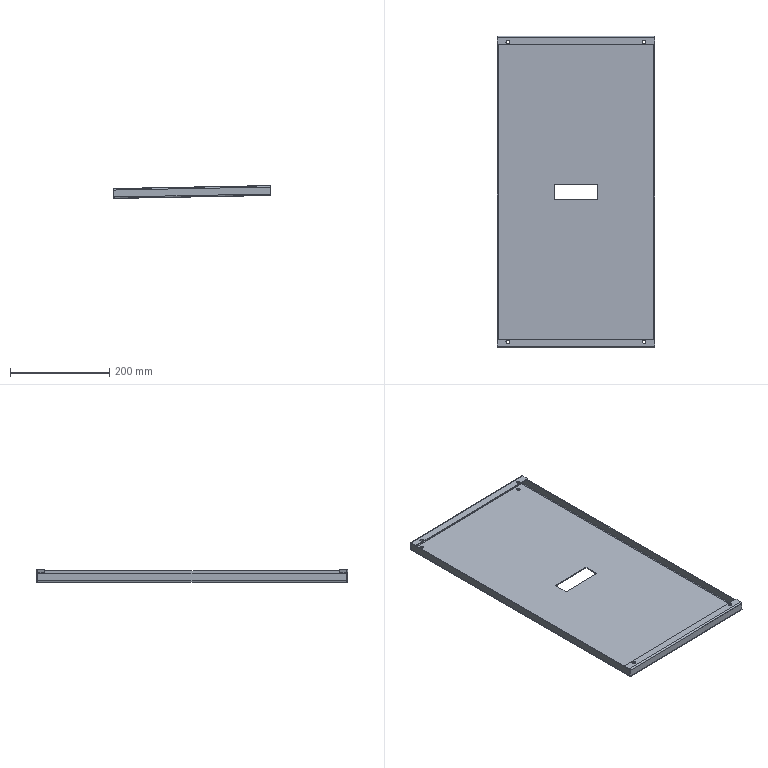Component | SolidWorks | 02FrameEndPlate1-2 | 1 solid | 78 faces | volume 470626 mm3 | plane 50 | cylinder 28 | commonest cylinder face diameters 7 x16 6 x6 2 x6 | material A3 Steel